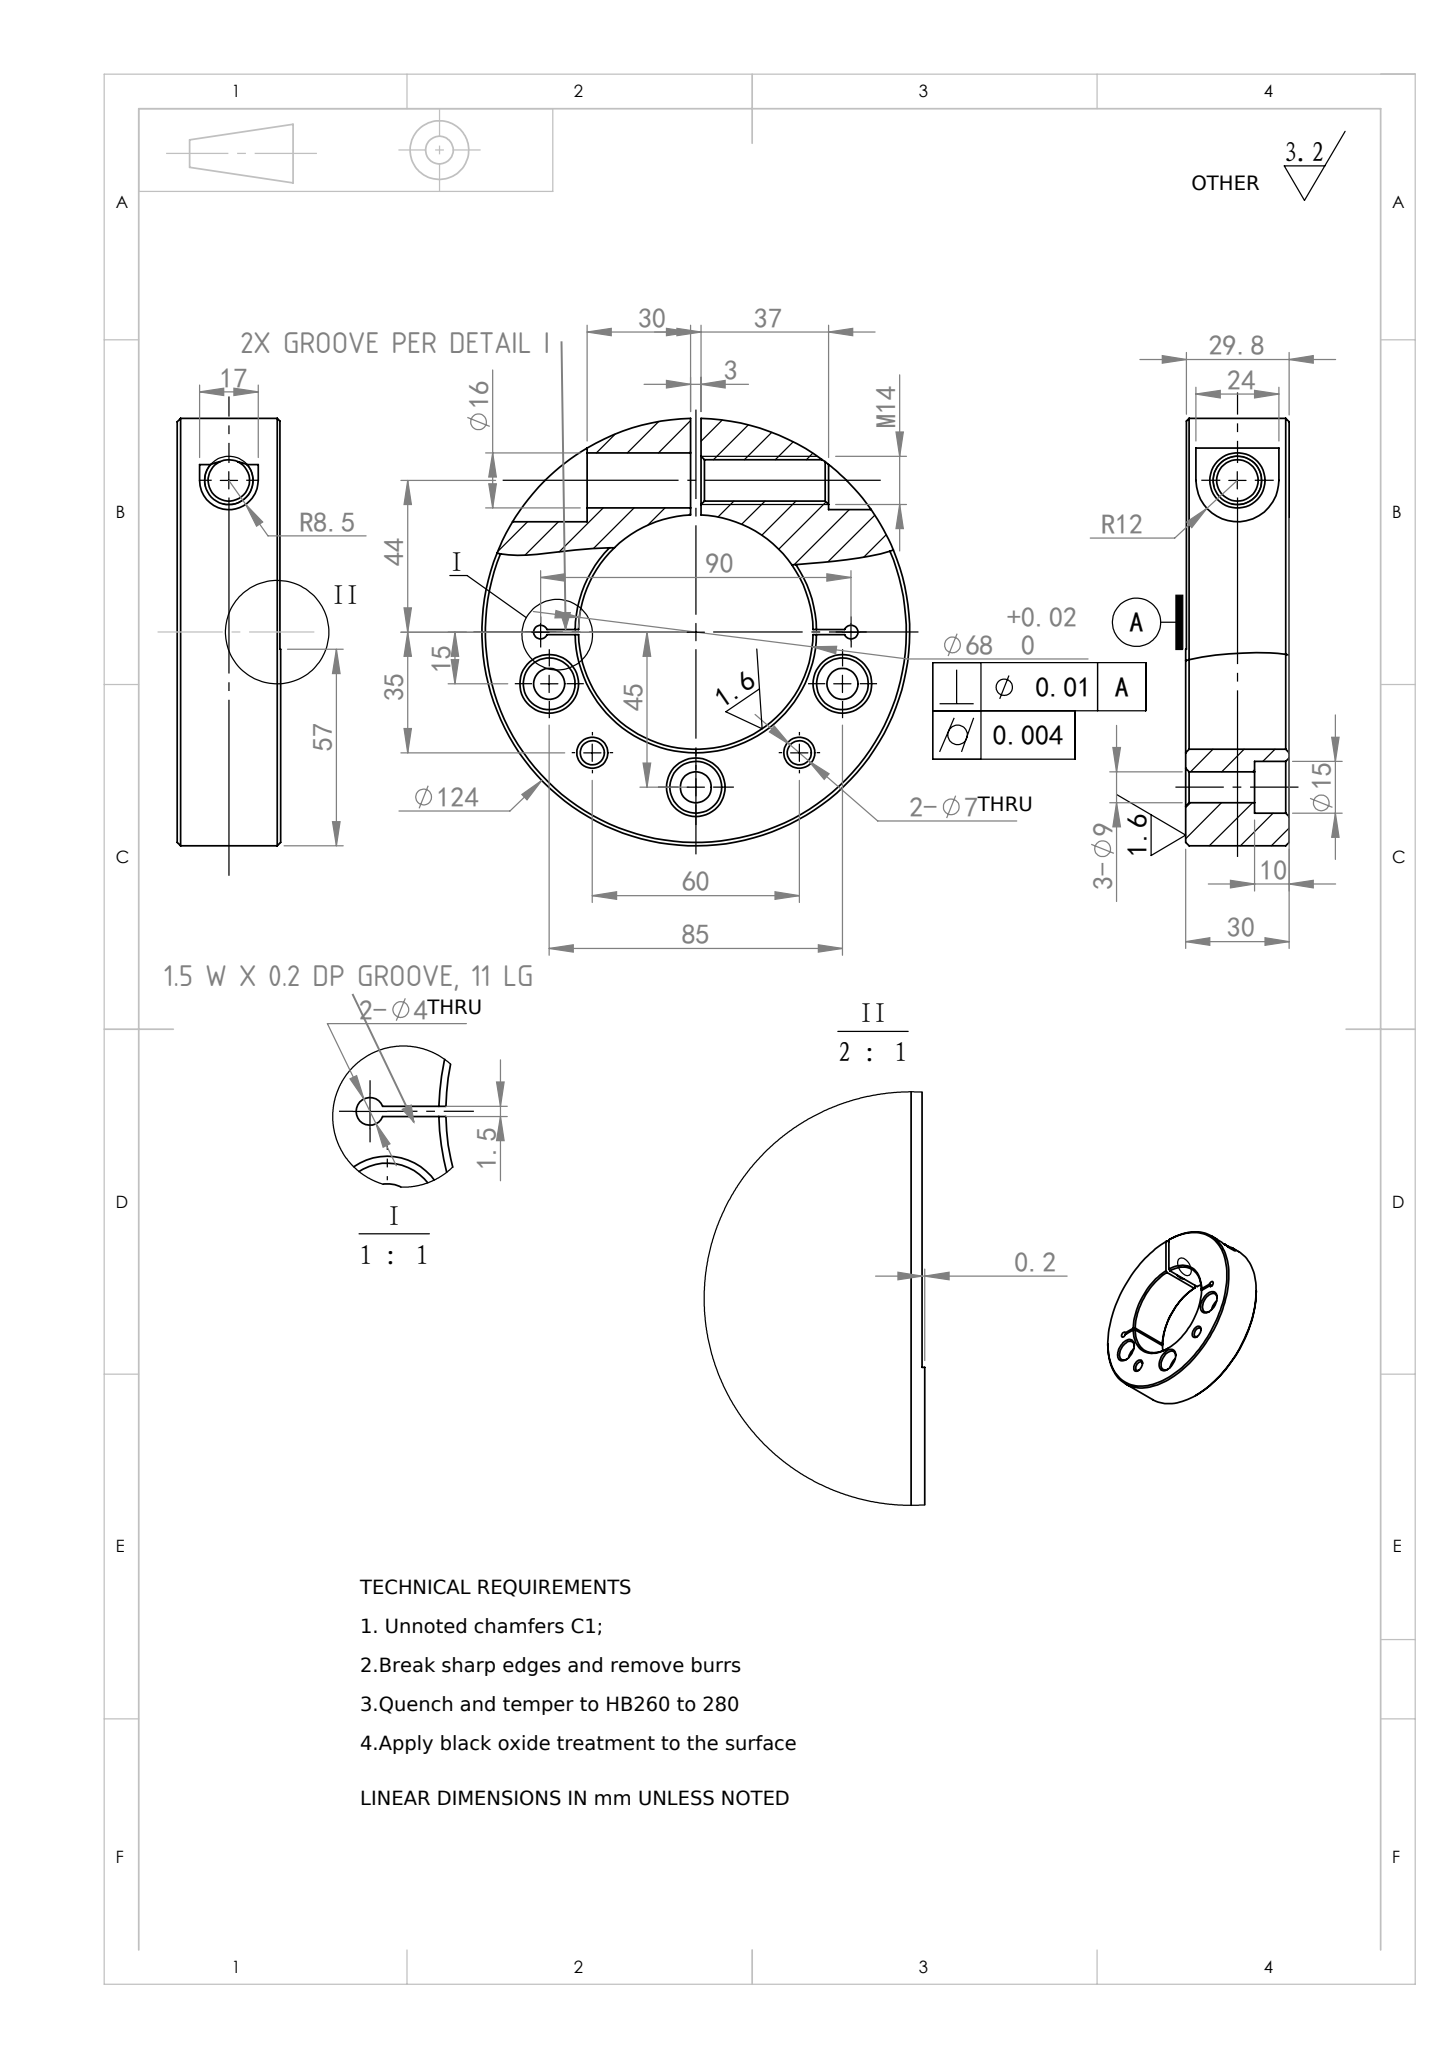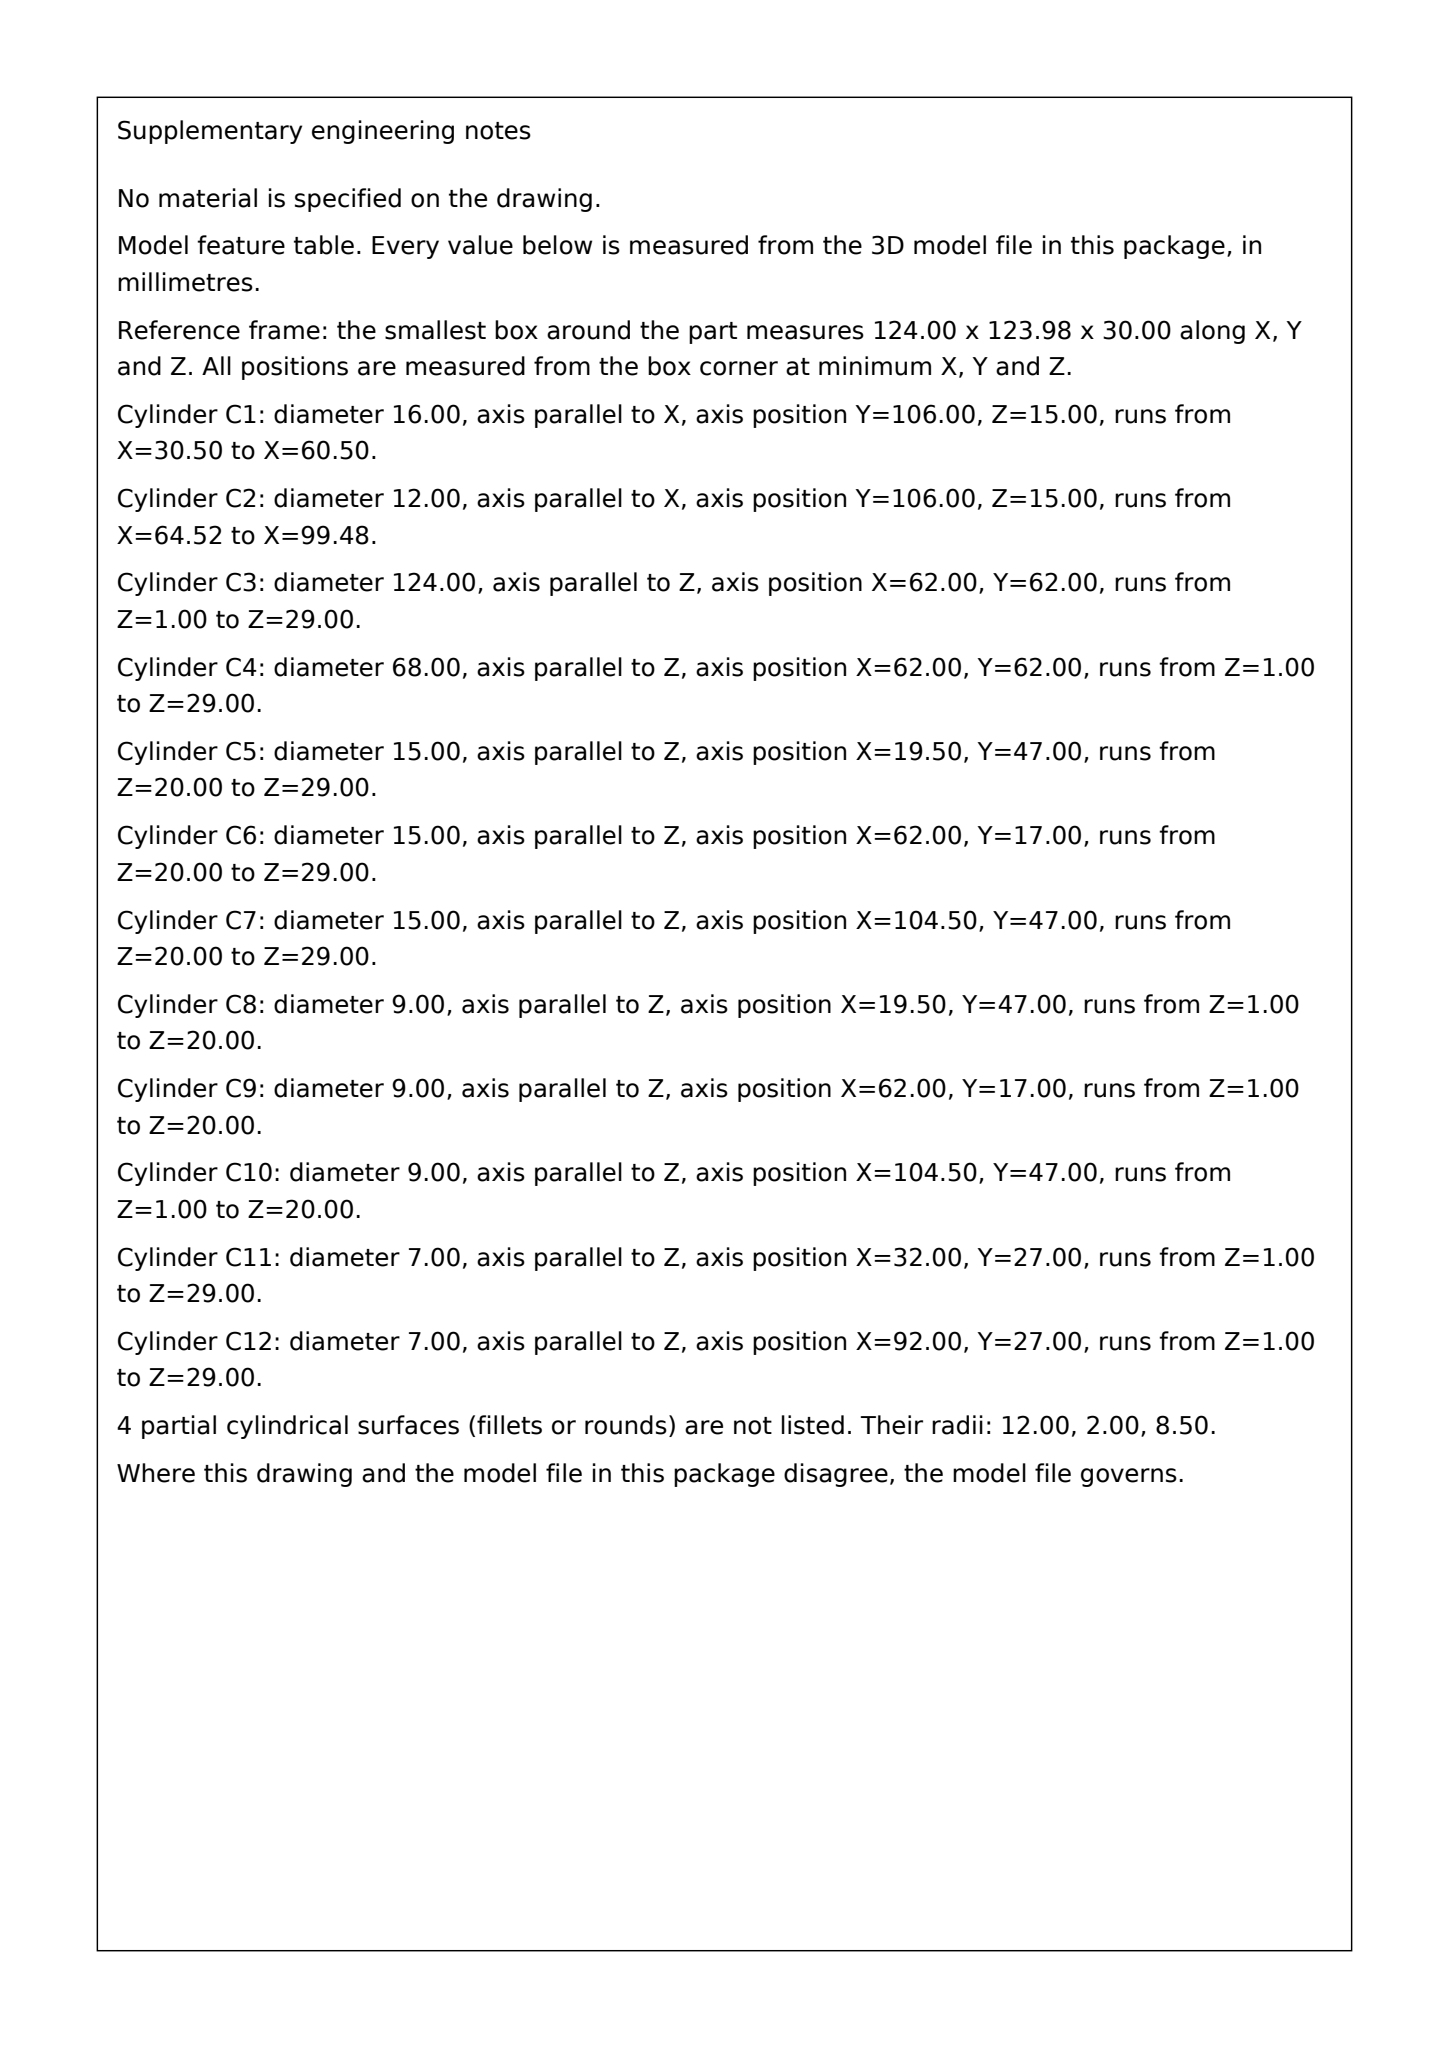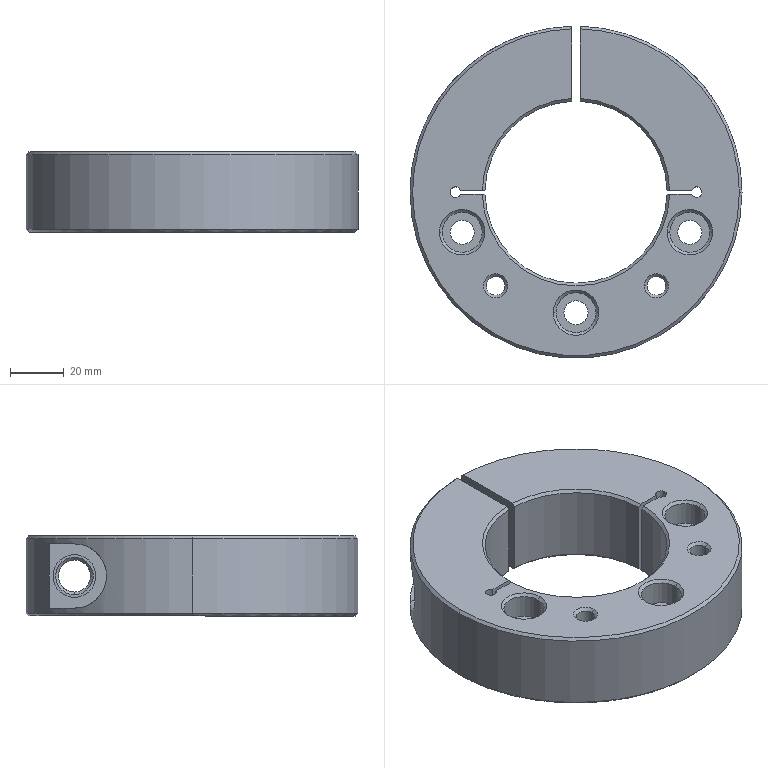Part | SolidWorks | mm | 1 solid | 89 faces | box 124 x 123.98 x 30 mm | volume 219578 mm3 | cone 37 | cylinder 31 | plane 21 | commonest cylinder face diameters 9 x6 15 x6 7 x4 4 x3 124 x3 68 x3 12 x2 16 x2
Drawing notes:
DETAIL I GROOVE: 1.5 W x 0.2 DP, Ø68 BORE TO Ø4 HOLE CL, 11 LG | from the solid: y-planes 61.25 & 62.75 (1.5 wide) with z-planes 0.0/0.2 (0.2 deep); Ø4 holes at x=17 & x=107, y=62; Ø68 bore at (62,62) -> 45-34=11 radial length
GROOVE PER DETAIL I ON FACE OPP Ø15 CBORES, 2 PL | from the solid: groove faces at z=0.2 from z=0 face; Ø15 cbores open at z=30 with bottoms at z=20 (count 3)
build123d program:
from build123d import *

# Parameters (mm, degrees)
EXTRUDE1_DEPTH                                  = 15
M8_HEX_SOCKET_HEAD_CAP_SCREW_CBORE1_D           = 9
M8_HEX_SOCKET_HEAD_CAP_SCREW_CBORE1_CBORE_D     = 15
M8_HEX_SOCKET_HEAD_CAP_SCREW_CBORE1_CBORE_DEPTH = 10
F_7_0_7_DIAMETER_HOLE1_AT_2_COUNT               = 2
F_7_0_7_DIAMETER_HOLE1_AT_2_PITCH               = 60
CUT_EXTRUDE1_START                              = -31.5
CUT_EXTRUDE1_DEPTH                              = 30
CUT_EXTRUDE2_REACH                              = 115.187
SKETCH7_R                                       = 8
CUT_EXTRUDE3_START                              = 38.5
CUT_EXTRUDE3_DEPTH                              = 20
CHAMFER1_SIZE                                   = 1
SKETCH11_W                                      = 5
SKETCH11_H                                      = 75
CUT_EXTRUDE4_DEPTH                              = 75


with BuildPart() as part:
    # Sketch1 → Extrude1 (new, symmetric)
    with BuildSketch(Plane.XY):
        with BuildLine():
            Line((-1.5, 61.982), (-1.5, 33.967))
            ThreePointArc((-1.5, 33.967), (-24.305, 23.775), (-33.992, 0.75))
            Line((-33.992, 0.75), (-43.146, 0.75))
            ThreePointArc((-43.146, 0.75), (-47, 0), (-43.146, -0.75))
            Line((-43.146, -0.75), (-33.992, -0.75))
            ThreePointArc((-33.992, -0.75), (0, -34), (33.992, -0.75))
            Line((33.992, -0.75), (43.146, -0.75))
            ThreePointArc((43.146, -0.75), (47, 0), (43.146, 0.75))
            Line((43.146, 0.75), (33.992, 0.75))
            ThreePointArc((33.992, 0.75), (24.305, 23.775), (1.5, 33.967))
            Line((1.5, 33.967), (1.5, 61.982))
            ThreePointArc((1.5, 61.982), (0, -62), (-1.5, 61.982))
        make_face()
    extrude(amount=EXTRUDE1_DEPTH, both=True)

    # M8 Hex Socket Head Cap Screw CBORE1 (through all)
    with Locations(Plane.XY.offset(15)):
        with Locations((-42.5, -15), (42.5, -15), (0, -45)):
            CounterBoreHole(M8_HEX_SOCKET_HEAD_CAP_SCREW_CBORE1_D / 2, M8_HEX_SOCKET_HEAD_CAP_SCREW_CBORE1_CBORE_D / 2, M8_HEX_SOCKET_HEAD_CAP_SCREW_CBORE1_CBORE_DEPTH)

    # Sketch4 → 7.0 _7_ Diameter Hole1 (revolve, cut)
    with BuildSketch(Plane(origin=(-30, -35, 15), x_dir=(0, -1, 0), z_dir=(1, 0, 0))):
        Polygon((0, 0), (0, 30), (4.5, 30), (3.5, 29), (3.5, 1), (4.5, 0), align=None)
    f_7_0_7_diameter_hole1 = revolve(axis=Axis((-30, -35, 21.35), (0, 0, -1)), mode=Mode.SUBTRACT)

    # 7.0 _7_ Diameter Hole1 at 2: 7.0 _7_ Diameter Hole1 ×2
    with Locations(*[(i * F_7_0_7_DIAMETER_HOLE1_AT_2_PITCH, 0, 0) for i in range(1, F_7_0_7_DIAMETER_HOLE1_AT_2_COUNT)]):
        add(f_7_0_7_diameter_hole1, mode=Mode.SUBTRACT)

    # Sketch6 → Cut-Extrude1 (cut)
    with BuildSketch(Plane(origin=(0, 0, 0), x_dir=(0, 0, -1), z_dir=(1, 0, 0)).offset(CUT_EXTRUDE1_START)):
        with BuildLine():
            Line((-12, 44), (-12, 61.982))
            Line((-12, 61.982), (12, 61.982))
            Line((12, 61.982), (12, 44))
            ThreePointArc((12, 44), (0, 32), (-12, 44))
        make_face()
    extrude(amount=-CUT_EXTRUDE1_DEPTH, mode=Mode.SUBTRACT)

    # Sketch7 → Cut-Extrude2 (cut, up to next)
    with BuildSketch(Plane.ZY.offset(31.5), mode=Mode.PRIVATE) as cut_extrude2_sk1:
        with Locations((0, 44)):
            Circle(SKETCH7_R)
    cut_extrude2_tool1 = extrude(cut_extrude2_sk1.sketch, amount=-CUT_EXTRUDE2_REACH, mode=Mode.PRIVATE) & part.part
    add(cut_extrude2_tool1.solids().sort_by_distance((-31.5, 44, 0))[0], mode=Mode.SUBTRACT)

    # Sketch8 → Cut-Extrude3 (cut)
    with BuildSketch(Plane(origin=(0, 0, 0), x_dir=(0, 0, -1), z_dir=(1, 0, 0)).offset(CUT_EXTRUDE3_START)):
        with BuildLine():
            Line((-8.5, 44), (-8.5, 61.982))
            Line((-8.5, 61.982), (8.5, 61.982))
            Line((8.5, 61.982), (8.5, 44))
            ThreePointArc((8.5, 44), (0, 35.5), (-8.5, 44))
        make_face()
    extrude(amount=CUT_EXTRUDE3_DEPTH, mode=Mode.SUBTRACT)

    # Sketch9 → M14 Tapped Hole1 (revolve, cut)
    with BuildSketch(Plane(origin=(1.5, 44, 0), x_dir=(0, 0, 1), z_dir=(0, 1, 0))):
        Polygon((0, 0), (0, 37), (7.025, 37), (6, 35.975), (6, 1.025), (7.025, 0), align=None)
    revolve(axis=Axis((-4.85, 44, 0), (1, 0, 0)), mode=Mode.SUBTRACT)

    # Chamfer1
    chamfer1_edges = [part.edges().sort_by_distance(p)[0] for p in [
        (24.305, 23.775, 15),
        (-24.305, 23.775, -15),
        (0, -34, -15),
        (24.305, 23.775, -15),
        (0, -62, -15),
        (0, -34, 15),
        (-24.305, 23.775, 15),
        (-7.5, -45, 15),
        (4.5, -45, -15),
        (0, -62, 15),
        (35, -15, 15),
        (47, -15, -15),
        (-50, -15, 15),
        (-38, -15, -15),
    ]]
    chamfer(chamfer1_edges, length=CHAMFER1_SIZE)

    # Sketch11 → Cut-Extrude4 (cut, symmetric)
    with BuildSketch(Plane(origin=(0, 0, 0), x_dir=(0, 0, -1), z_dir=(1, 0, 0))):
        with Locations((17.3, 32.5)):
            Rectangle(SKETCH11_W, SKETCH11_H)
    extrude(amount=CUT_EXTRUDE4_DEPTH, both=True, mode=Mode.SUBTRACT)


solid = part.part